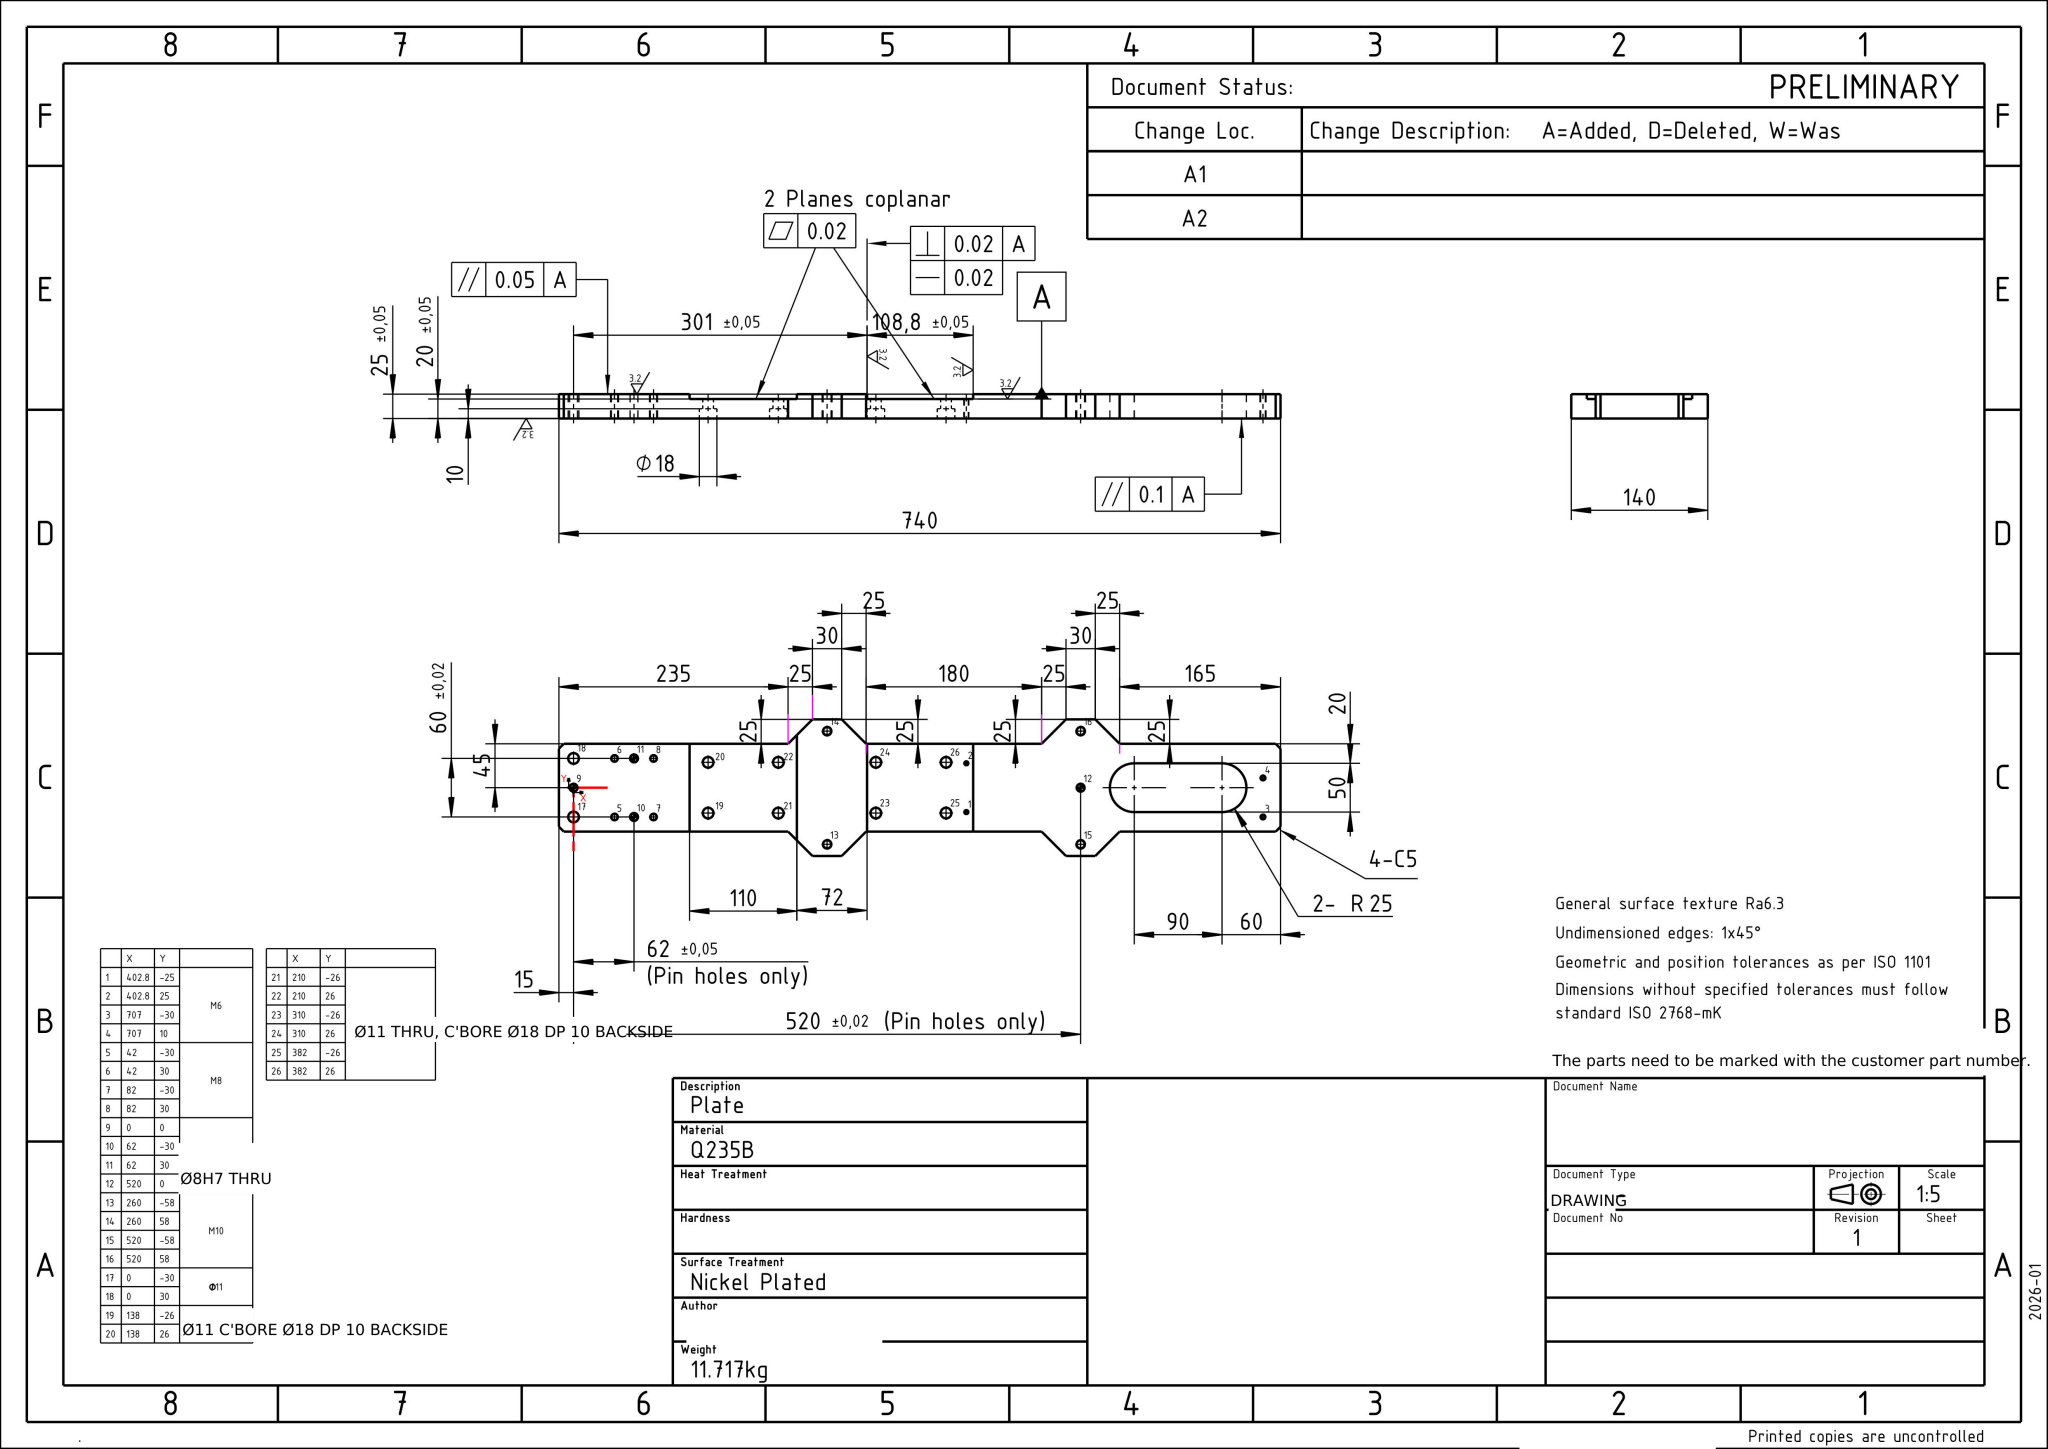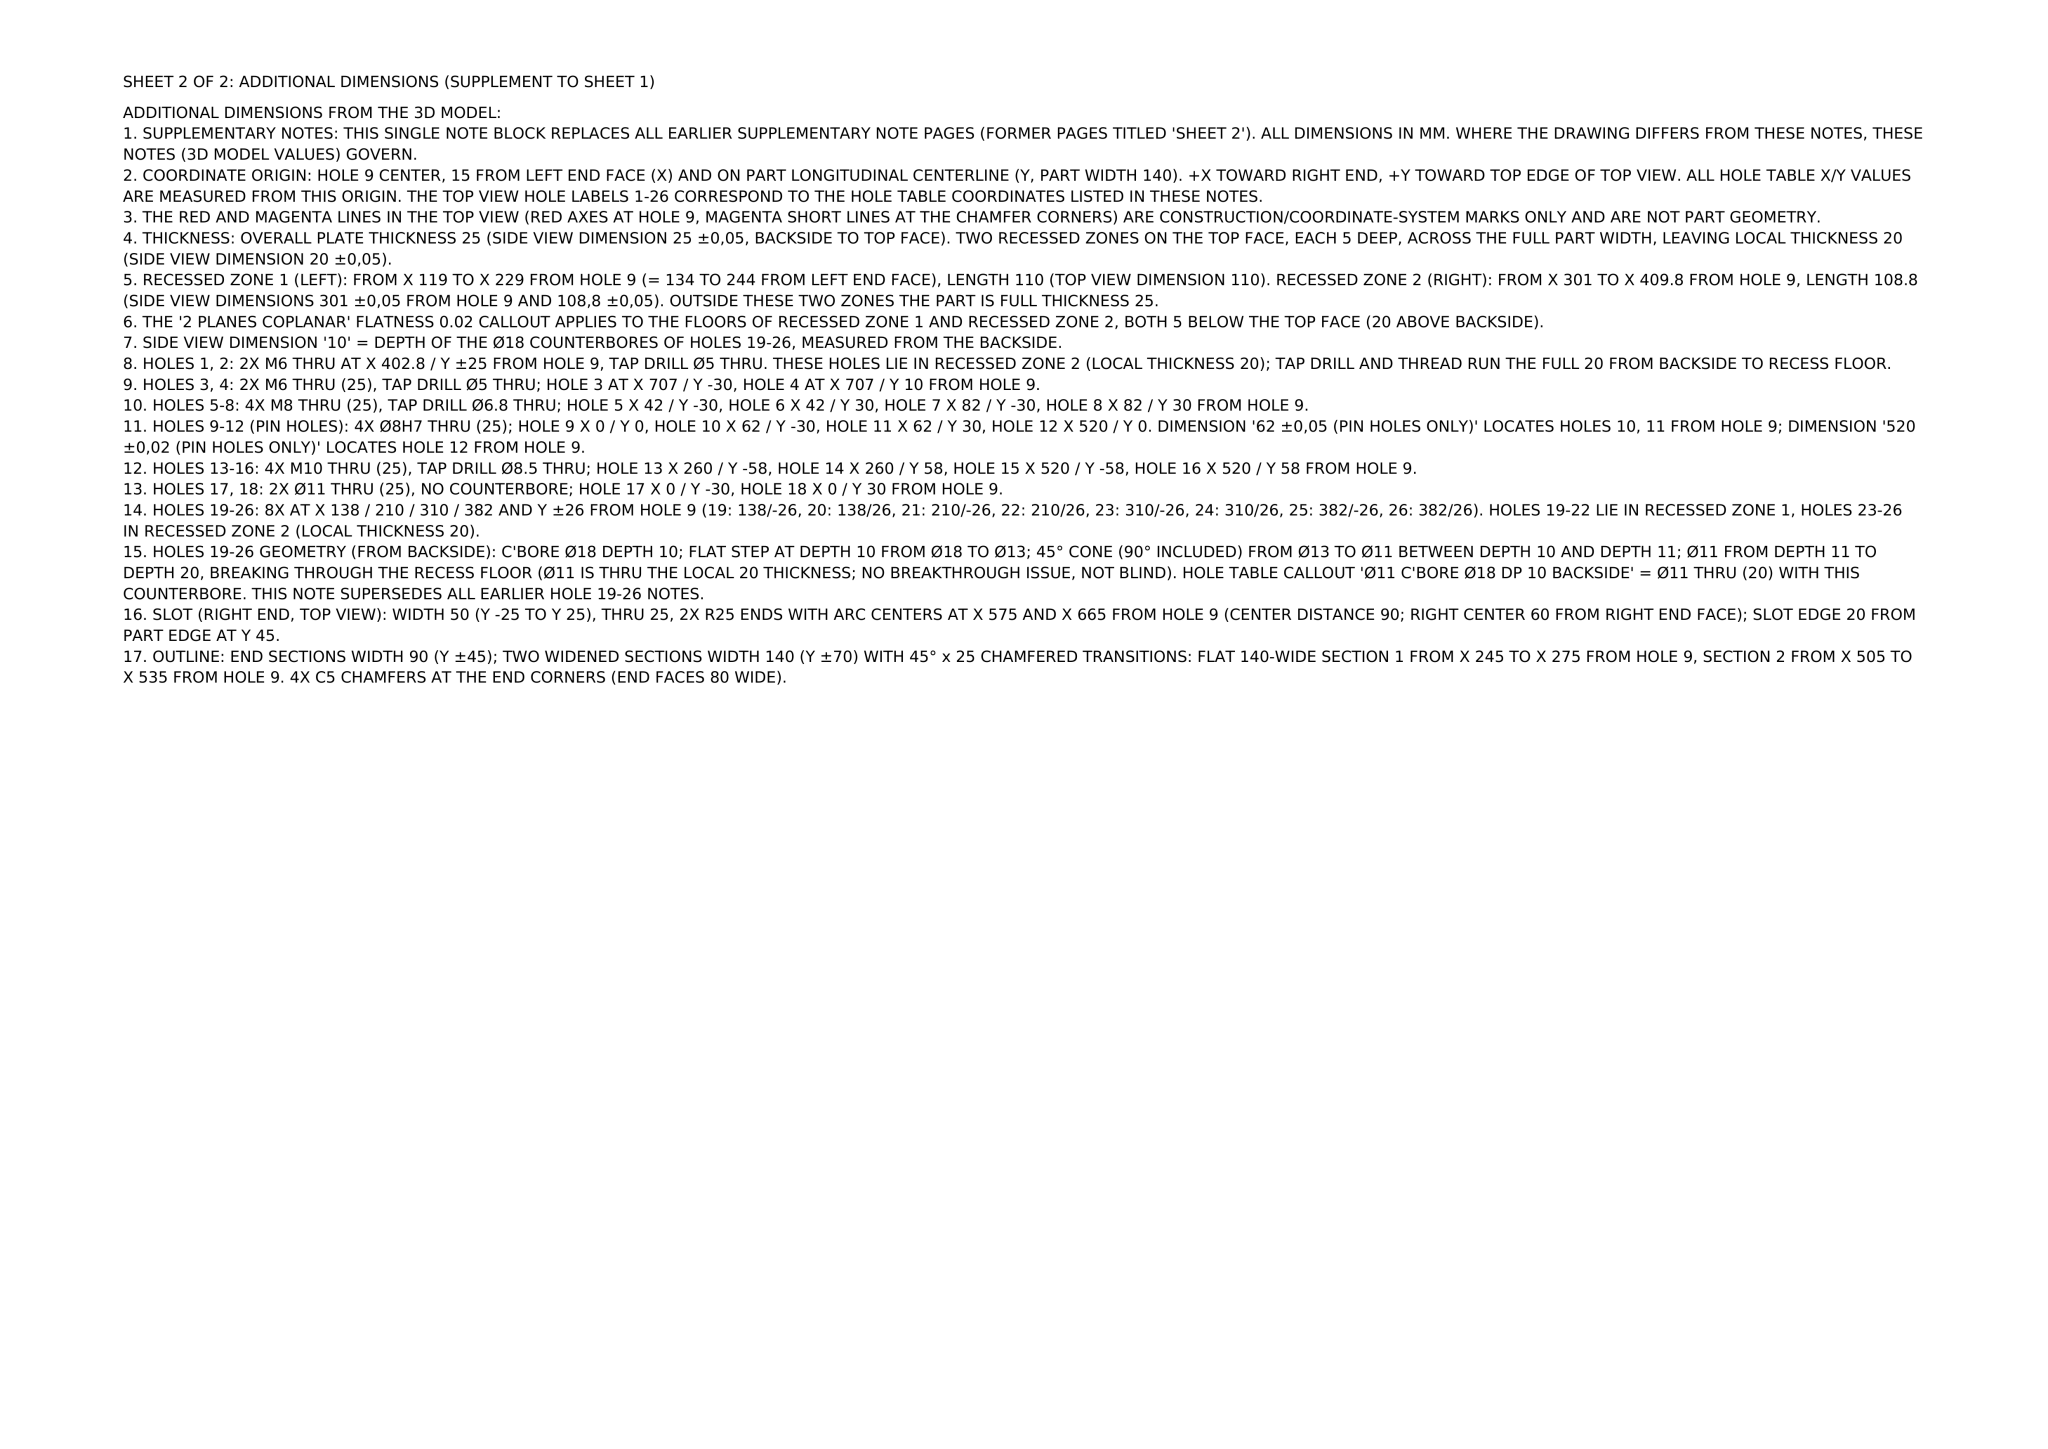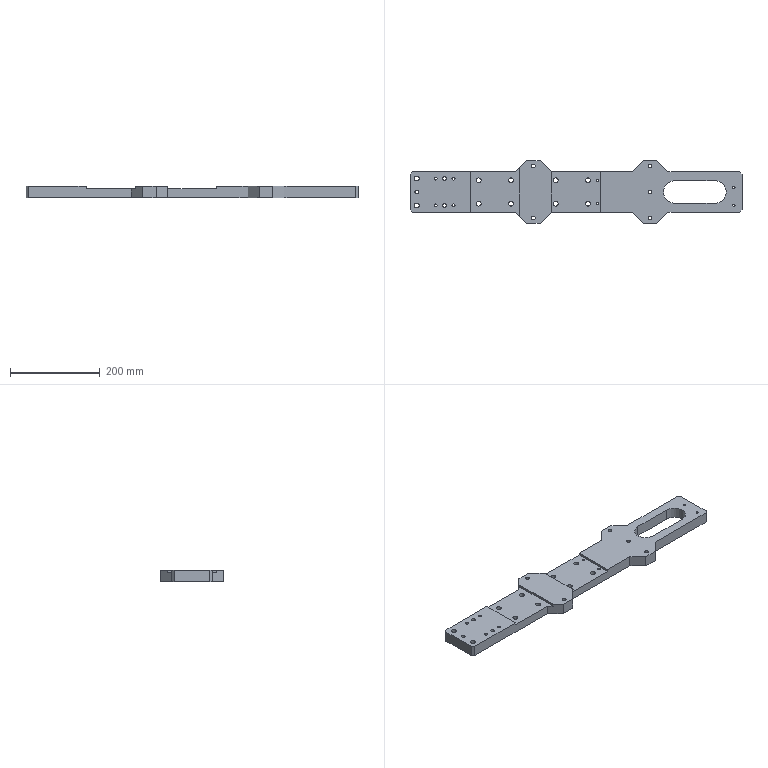Part | NX | mm | 1 solid | 88 faces | box 740 x 140 x 25 mm | volume 1491839 mm3 | plane 44 | cylinder 36 | cone 8 | commonest cylinder face diameters 11 x10 18 x8 5 x4 6.8 x4 8 x4 8.5 x4 50 x2